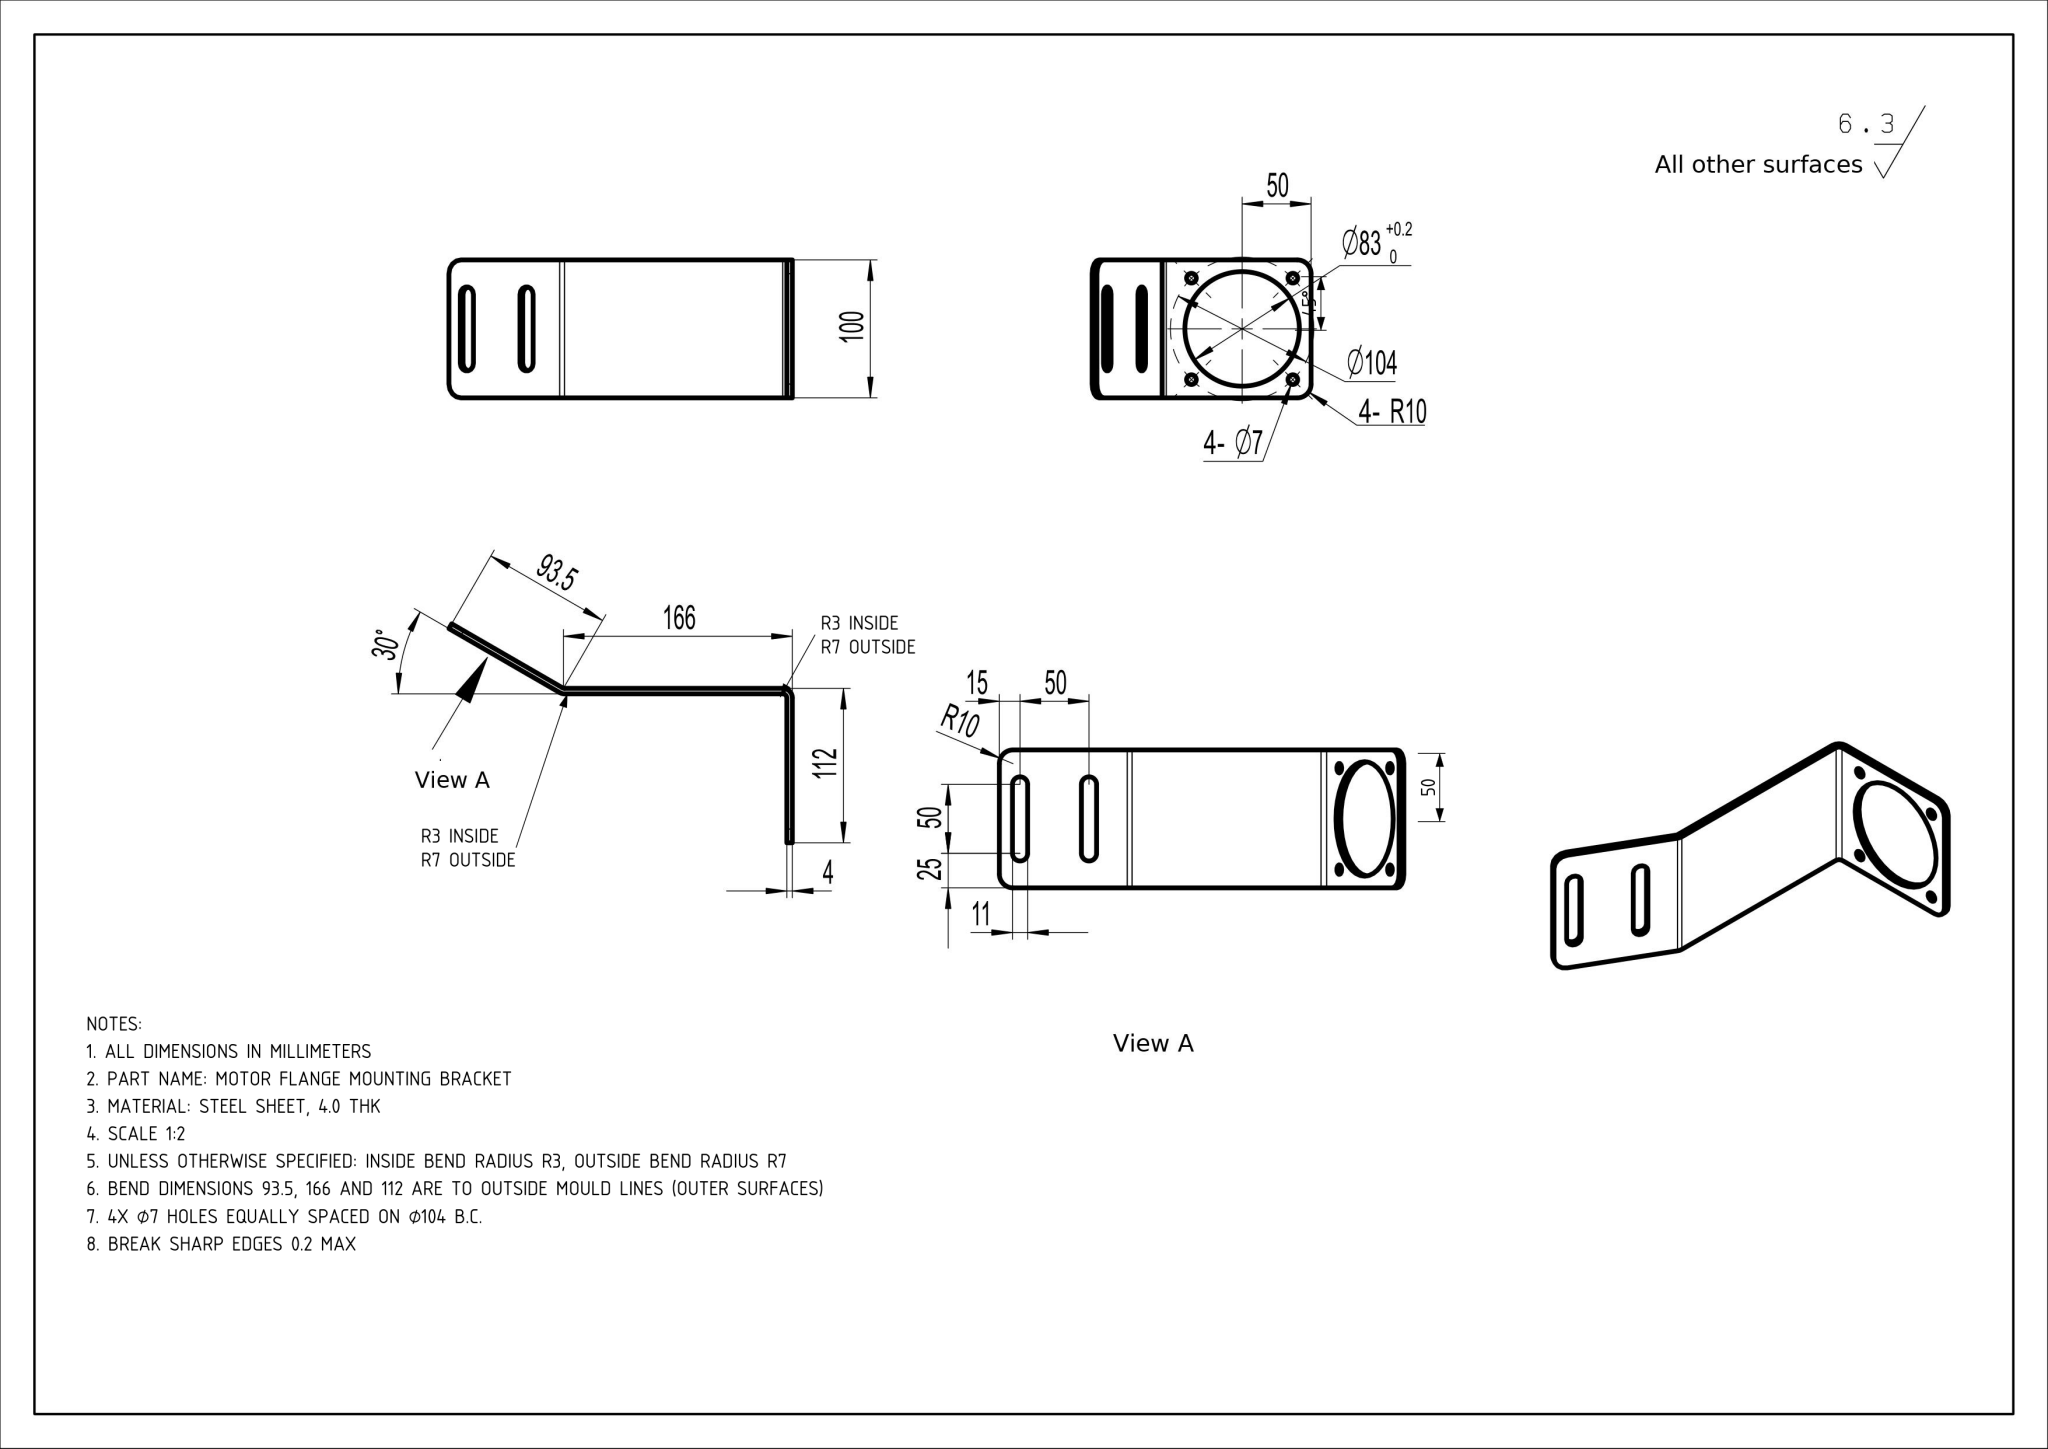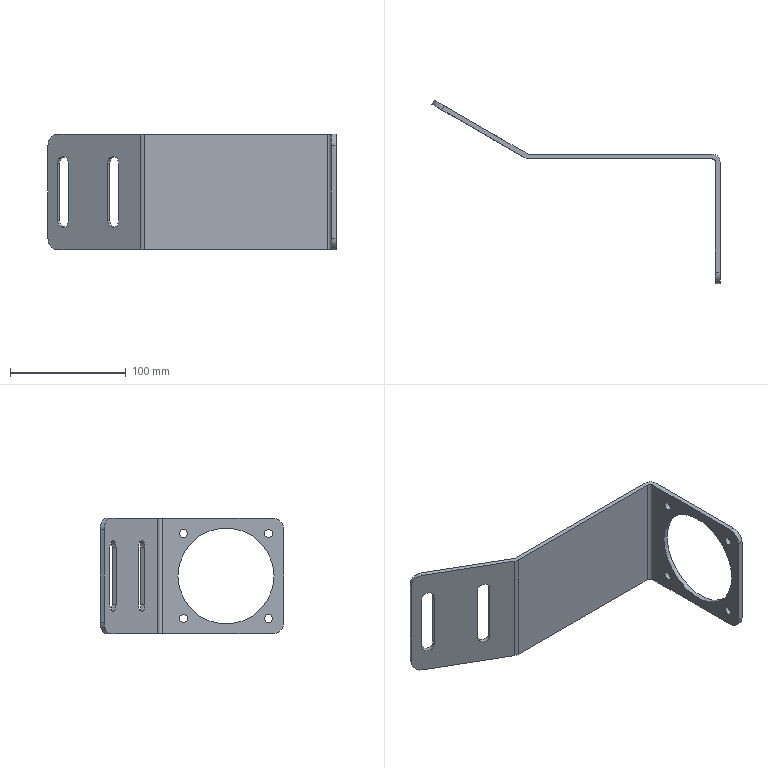Part | NX | mm | 1 solid | 31 faces | box 249.03 x 158.77 x 100 mm | volume 118808 mm3 | cylinder 17 | plane 14 | commonest cylinder face diameters 7 x4 11 x4 20 x4 14 x2 6 x2 83 x1
STEP:
#1=CARTESIAN_POINT('',(0.,0.,0.));
#2=DIRECTION('',(0.,0.,1.));
#3=DIRECTION('',(1.,0.,0.));
#4=AXIS2_PLACEMENT_3D('',#1,#2,#3);
#5=(LENGTH_UNIT()NAMED_UNIT(*)SI_UNIT(.MILLI.,.METRE.));
#6=UNCERTAINTY_MEASURE_WITH_UNIT(LENGTH_MEASURE(0.00002),#5,'','');
#7=(NAMED_UNIT(*)PLANE_ANGLE_UNIT()SI_UNIT($,.RADIAN.));
#8=PLANE_ANGLE_MEASURE_WITH_UNIT(PLANE_ANGLE_MEASURE(0.01745),#7);
#9=DIMENSIONAL_EXPONENTS(0.,0.,0.,0.,0.,0.,0.);
#10=(CONVERSION_BASED_UNIT('',#8)NAMED_UNIT(#9)PLANE_ANGLE_UNIT());
#11=(NAMED_UNIT(*)SI_UNIT($,.STERADIAN.)SOLID_ANGLE_UNIT());
#12=(GEOMETRIC_REPRESENTATION_CONTEXT(3)GLOBAL_UNCERTAINTY_ASSIGNED_CONTEXT((#6))GLOBAL_UNIT_ASSIGNED_CONTEXT((#5,#10,#11))REPRESENTATION_CONTEXT('',''));
#13=SHAPE_REPRESENTATION('',(#4),#12);
#14=CARTESIAN_POINT('',(4.,10.,0.));
#15=VERTEX_POINT('',#14);
#16=CARTESIAN_POINT('',(4.,105.,0.));
#17=VERTEX_POINT('',#16);
#18=CARTESIAN_POINT('',(4.,0.,0.));
#19=DIRECTION('',(0.,1.,0.));
#20=VECTOR('',#19,1.);
#21=LINE('',#18,#20);
#22=EDGE_CURVE('',#15,#17,#21,.T.);
#23=ORIENTED_EDGE('',*,*,#22,.F.);
#24=CARTESIAN_POINT('',(0.,10.,0.));
#25=VERTEX_POINT('',#24);
#26=CARTESIAN_POINT('',(4.,10.,0.));
#27=DIRECTION('',(-1.,0.,0.));
#28=VECTOR('',#27,1.);
#29=LINE('',#26,#28);
#30=EDGE_CURVE('',#15,#25,#29,.T.);
#31=ORIENTED_EDGE('',*,*,#30,.T.);
#32=CARTESIAN_POINT('',(0.,105.,0.));
#33=VERTEX_POINT('',#32);
#34=CARTESIAN_POINT('',(0.,0.,0.));
#35=DIRECTION('',(0.,1.,0.));
#36=VECTOR('',#35,1.);
#37=LINE('',#34,#36);
#38=EDGE_CURVE('',#25,#33,#37,.T.);
#39=ORIENTED_EDGE('',*,*,#38,.T.);
#40=CARTESIAN_POINT('',(-3.,108.,0.));
#41=VERTEX_POINT('',#40);
#42=CARTESIAN_POINT('',(-3.,105.,0.));
#43=DIRECTION('',(0.,0.,1.));
#44=DIRECTION('',(1.,0.,0.));
#45=AXIS2_PLACEMENT_3D('',#42,#43,#44);
#46=CIRCLE('',#45,3.);
#47=EDGE_CURVE('',#33,#41,#46,.T.);
#48=ORIENTED_EDGE('',*,*,#47,.T.);
#49=CARTESIAN_POINT('',(-161.214,108.,0.));
#50=VERTEX_POINT('',#49);
#51=CARTESIAN_POINT('',(108.786,108.,0.));
#52=DIRECTION('',(-1.,0.,0.));
#53=VECTOR('',#52,1.);
#54=LINE('',#51,#53);
#55=EDGE_CURVE('',#41,#50,#54,.T.);
#56=ORIENTED_EDGE('',*,*,#55,.T.);
#57=CARTESIAN_POINT('',(-164.714,108.938,0.));
#58=VERTEX_POINT('',#57);
#59=CARTESIAN_POINT('',(-161.214,115.,0.));
#60=DIRECTION('',(0.,-0.,-1.));
#61=DIRECTION('',(0.,1.,0.));
#62=AXIS2_PLACEMENT_3D('',#59,#60,#61);
#63=CIRCLE('',#62,7.);
#64=EDGE_CURVE('',#50,#58,#63,.T.);
#65=ORIENTED_EDGE('',*,*,#64,.T.);
#66=CARTESIAN_POINT('',(-236.367,150.307,0.));
#67=VERTEX_POINT('',#66);
#68=CARTESIAN_POINT('',(71.072,-27.193,0.));
#69=DIRECTION('',(-0.866,0.5,0.));
#70=VECTOR('',#69,1.);
#71=LINE('',#68,#70);
#72=EDGE_CURVE('',#58,#67,#71,.T.);
#73=ORIENTED_EDGE('',*,*,#72,.T.);
#74=CARTESIAN_POINT('',(-234.367,153.771,0.));
#75=VERTEX_POINT('',#74);
#76=CARTESIAN_POINT('',(-241.36,141.659,0.));
#77=DIRECTION('',(0.5,0.866,0.));
#78=VECTOR('',#77,1.);
#79=LINE('',#76,#78);
#80=EDGE_CURVE('',#67,#75,#79,.T.);
#81=ORIENTED_EDGE('',*,*,#80,.T.);
#82=CARTESIAN_POINT('',(-162.714,112.402,0.));
#83=VERTEX_POINT('',#82);
#84=CARTESIAN_POINT('',(73.072,-23.729,0.));
#85=DIRECTION('',(-0.866,0.5,0.));
#86=VECTOR('',#85,1.);
#87=LINE('',#84,#86);
#88=EDGE_CURVE('',#83,#75,#87,.T.);
#89=ORIENTED_EDGE('',*,*,#88,.F.);
#90=CARTESIAN_POINT('',(-161.214,112.,0.));
#91=VERTEX_POINT('',#90);
#92=CARTESIAN_POINT('',(-161.214,115.,0.));
#93=DIRECTION('',(0.,-0.,-1.));
#94=DIRECTION('',(-1.,0.,-0.));
#95=AXIS2_PLACEMENT_3D('',#92,#93,#94);
#96=CIRCLE('',#95,3.);
#97=EDGE_CURVE('',#91,#83,#96,.T.);
#98=ORIENTED_EDGE('',*,*,#97,.F.);
#99=CARTESIAN_POINT('',(-3.,112.,0.));
#100=VERTEX_POINT('',#99);
#101=CARTESIAN_POINT('',(108.786,112.,0.));
#102=DIRECTION('',(-1.,0.,0.));
#103=VECTOR('',#102,1.);
#104=LINE('',#101,#103);
#105=EDGE_CURVE('',#100,#91,#104,.T.);
#106=ORIENTED_EDGE('',*,*,#105,.F.);
#107=CARTESIAN_POINT('',(-3.,105.,0.));
#108=DIRECTION('',(0.,0.,1.));
#109=DIRECTION('',(-1.,0.,0.));
#110=AXIS2_PLACEMENT_3D('',#107,#108,#109);
#111=CIRCLE('',#110,7.);
#112=EDGE_CURVE('',#17,#100,#111,.T.);
#113=ORIENTED_EDGE('',*,*,#112,.F.);
#114=EDGE_LOOP('',(#23,#31,#39,#48,#56,#65,#73,#81,#89,#98,#106,#113));
#115=FACE_OUTER_BOUND('',#114,.T.);
#116=CARTESIAN_POINT('',(4.,0.,0.));
#117=DIRECTION('',(0.,0.,1.));
#118=DIRECTION('',(1.,0.,0.));
#119=AXIS2_PLACEMENT_3D('',#116,#117,#118);
#120=PLANE('',#119);
#121=ADVANCED_FACE('',(#115),#120,.F.);
#122=ORIENTED_EDGE('',*,*,#105,.T.);
#123=CARTESIAN_POINT('',(-161.214,112.,100.));
#124=VERTEX_POINT('',#123);
#125=CARTESIAN_POINT('',(-161.214,112.,-19.));
#126=DIRECTION('',(0.,0.,1.));
#127=VECTOR('',#126,1.);
#128=LINE('',#125,#127);
#129=EDGE_CURVE('',#91,#124,#128,.T.);
#130=ORIENTED_EDGE('',*,*,#129,.T.);
#131=CARTESIAN_POINT('',(-3.,112.,100.));
#132=VERTEX_POINT('',#131);
#133=CARTESIAN_POINT('',(-291.214,112.,100.));
#134=DIRECTION('',(1.,-0.,-0.));
#135=VECTOR('',#134,1.);
#136=LINE('',#133,#135);
#137=EDGE_CURVE('',#124,#132,#136,.T.);
#138=ORIENTED_EDGE('',*,*,#137,.T.);
#139=CARTESIAN_POINT('',(-3.,112.,-30.));
#140=DIRECTION('',(0.,-0.,1.));
#141=VECTOR('',#140,1.);
#142=LINE('',#139,#141);
#143=EDGE_CURVE('',#100,#132,#142,.T.);
#144=ORIENTED_EDGE('',*,*,#143,.F.);
#145=EDGE_LOOP('',(#122,#130,#138,#144));
#146=FACE_OUTER_BOUND('',#145,.T.);
#147=CARTESIAN_POINT('',(58.786,112.,50.));
#148=DIRECTION('',(0.,1.,0.));
#149=DIRECTION('',(0.,0.,-1.));
#150=AXIS2_PLACEMENT_3D('',#147,#148,#149);
#151=PLANE('',#150);
#152=ADVANCED_FACE('',(#146),#151,.T.);
#153=CARTESIAN_POINT('',(4.,83.27,13.23));
#154=VERTEX_POINT('',#153);
#155=CARTESIAN_POINT('',(4.,86.77,13.23));
#156=DIRECTION('',(1.,0.,0.));
#157=DIRECTION('',(0.,-1.,0.));
#158=AXIS2_PLACEMENT_3D('',#155,#156,#157);
#159=CIRCLE('',#158,3.5);
#160=EDGE_CURVE('',#154,#154,#159,.T.);
#161=ORIENTED_EDGE('',*,*,#160,.F.);
#162=EDGE_LOOP('',(#161));
#163=FACE_BOUND('',#162,.T.);
#164=CARTESIAN_POINT('',(4.,16.73,86.77));
#165=VERTEX_POINT('',#164);
#166=CARTESIAN_POINT('',(4.,13.23,86.77));
#167=DIRECTION('',(1.,0.,0.));
#168=DIRECTION('',(0.,1.,0.));
#169=AXIS2_PLACEMENT_3D('',#166,#167,#168);
#170=CIRCLE('',#169,3.5);
#171=EDGE_CURVE('',#165,#165,#170,.T.);
#172=ORIENTED_EDGE('',*,*,#171,.F.);
#173=EDGE_LOOP('',(#172));
#174=FACE_BOUND('',#173,.T.);
#175=CARTESIAN_POINT('',(4.,13.23,16.73));
#176=VERTEX_POINT('',#175);
#177=CARTESIAN_POINT('',(4.,13.23,13.23));
#178=DIRECTION('',(1.,0.,0.));
#179=DIRECTION('',(0.,0.,1.));
#180=AXIS2_PLACEMENT_3D('',#177,#178,#179);
#181=CIRCLE('',#180,3.5);
#182=EDGE_CURVE('',#176,#176,#181,.T.);
#183=ORIENTED_EDGE('',*,*,#182,.F.);
#184=EDGE_LOOP('',(#183));
#185=FACE_BOUND('',#184,.T.);
#186=CARTESIAN_POINT('',(4.,86.77,83.27));
#187=VERTEX_POINT('',#186);
#188=CARTESIAN_POINT('',(4.,86.77,86.77));
#189=DIRECTION('',(1.,0.,0.));
#190=DIRECTION('',(0.,0.,-1.));
#191=AXIS2_PLACEMENT_3D('',#188,#189,#190);
#192=CIRCLE('',#191,3.5);
#193=EDGE_CURVE('',#187,#187,#192,.T.);
#194=ORIENTED_EDGE('',*,*,#193,.F.);
#195=EDGE_LOOP('',(#194));
#196=FACE_BOUND('',#195,.T.);
#197=CARTESIAN_POINT('',(4.,91.5,50.));
#198=VERTEX_POINT('',#197);
#199=CARTESIAN_POINT('',(4.,50.,50.));
#200=DIRECTION('',(1.,0.,0.));
#201=DIRECTION('',(0.,1.,0.));
#202=AXIS2_PLACEMENT_3D('',#199,#200,#201);
#203=CIRCLE('',#202,41.5);
#204=EDGE_CURVE('',#198,#198,#203,.T.);
#205=ORIENTED_EDGE('',*,*,#204,.F.);
#206=EDGE_LOOP('',(#205));
#207=FACE_BOUND('',#206,.T.);
#208=CARTESIAN_POINT('',(4.,0.,90.));
#209=VERTEX_POINT('',#208);
#210=CARTESIAN_POINT('',(4.,0.,10.));
#211=VERTEX_POINT('',#210);
#212=CARTESIAN_POINT('',(4.,0.,100.));
#213=DIRECTION('',(0.,-0.,-1.));
#214=VECTOR('',#213,1.);
#215=LINE('',#212,#214);
#216=EDGE_CURVE('',#209,#211,#215,.T.);
#217=ORIENTED_EDGE('',*,*,#216,.T.);
#218=CARTESIAN_POINT('',(4.,10.,10.));
#219=DIRECTION('',(1.,0.,0.));
#220=DIRECTION('',(0.,0.,-1.));
#221=AXIS2_PLACEMENT_3D('',#218,#219,#220);
#222=CIRCLE('',#221,10.);
#223=EDGE_CURVE('',#211,#15,#222,.T.);
#224=ORIENTED_EDGE('',*,*,#223,.T.);
#225=ORIENTED_EDGE('',*,*,#22,.T.);
#226=CARTESIAN_POINT('',(4.,105.,100.));
#227=VERTEX_POINT('',#226);
#228=CARTESIAN_POINT('',(4.,105.,-30.));
#229=DIRECTION('',(0.,0.,-1.));
#230=VECTOR('',#229,1.);
#231=LINE('',#228,#230);
#232=EDGE_CURVE('',#227,#17,#231,.T.);
#233=ORIENTED_EDGE('',*,*,#232,.F.);
#234=CARTESIAN_POINT('',(4.,10.,100.));
#235=VERTEX_POINT('',#234);
#236=CARTESIAN_POINT('',(4.,400.,100.));
#237=DIRECTION('',(0.,-1.,-0.));
#238=VECTOR('',#237,1.);
#239=LINE('',#236,#238);
#240=EDGE_CURVE('',#227,#235,#239,.T.);
#241=ORIENTED_EDGE('',*,*,#240,.T.);
#242=CARTESIAN_POINT('',(4.,10.,90.));
#243=DIRECTION('',(1.,0.,0.));
#244=DIRECTION('',(0.,0.,-1.));
#245=AXIS2_PLACEMENT_3D('',#242,#243,#244);
#246=CIRCLE('',#245,10.);
#247=EDGE_CURVE('',#235,#209,#246,.T.);
#248=ORIENTED_EDGE('',*,*,#247,.T.);
#249=EDGE_LOOP('',(#217,#224,#225,#233,#241,#248));
#250=FACE_BOUND('',#249,.T.);
#251=CARTESIAN_POINT('',(4.,50.,50.));
#252=DIRECTION('',(1.,0.,0.));
#253=DIRECTION('',(0.,0.,-1.));
#254=AXIS2_PLACEMENT_3D('',#251,#252,#253);
#255=PLANE('',#254);
#256=ADVANCED_FACE('',(#163,#174,#185,#196,#207,#250),#255,.T.);
#257=CARTESIAN_POINT('',(0.,0.,90.));
#258=VERTEX_POINT('',#257);
#259=CARTESIAN_POINT('',(0.,0.,10.));
#260=VERTEX_POINT('',#259);
#261=CARTESIAN_POINT('',(0.,0.,100.));
#262=DIRECTION('',(0.,-0.,-1.));
#263=VECTOR('',#262,1.);
#264=LINE('',#261,#263);
#265=EDGE_CURVE('',#258,#260,#264,.T.);
#266=ORIENTED_EDGE('',*,*,#265,.T.);
#267=CARTESIAN_POINT('',(4.,0.,10.));
#268=DIRECTION('',(1.,0.,0.));
#269=VECTOR('',#268,1.);
#270=LINE('',#267,#269);
#271=EDGE_CURVE('',#260,#211,#270,.T.);
#272=ORIENTED_EDGE('',*,*,#271,.T.);
#273=ORIENTED_EDGE('',*,*,#216,.F.);
#274=CARTESIAN_POINT('',(4.,0.,90.));
#275=DIRECTION('',(-1.,0.,0.));
#276=VECTOR('',#275,1.);
#277=LINE('',#274,#276);
#278=EDGE_CURVE('',#209,#258,#277,.T.);
#279=ORIENTED_EDGE('',*,*,#278,.T.);
#280=EDGE_LOOP('',(#266,#272,#273,#279));
#281=FACE_OUTER_BOUND('',#280,.T.);
#282=CARTESIAN_POINT('',(4.,0.,100.));
#283=DIRECTION('',(0.,1.,-0.));
#284=DIRECTION('',(0.,0.,1.));
#285=AXIS2_PLACEMENT_3D('',#282,#283,#284);
#286=PLANE('',#285);
#287=ADVANCED_FACE('',(#281),#286,.F.);
#288=CARTESIAN_POINT('',(0.,105.,100.));
#289=VERTEX_POINT('',#288);
#290=CARTESIAN_POINT('',(0.,10.,100.));
#291=VERTEX_POINT('',#290);
#292=CARTESIAN_POINT('',(0.,400.,100.));
#293=DIRECTION('',(0.,-1.,-0.));
#294=VECTOR('',#293,1.);
#295=LINE('',#292,#294);
#296=EDGE_CURVE('',#289,#291,#295,.T.);
#297=ORIENTED_EDGE('',*,*,#296,.T.);
#298=CARTESIAN_POINT('',(4.,10.,100.));
#299=DIRECTION('',(1.,0.,0.));
#300=VECTOR('',#299,1.);
#301=LINE('',#298,#300);
#302=EDGE_CURVE('',#291,#235,#301,.T.);
#303=ORIENTED_EDGE('',*,*,#302,.T.);
#304=ORIENTED_EDGE('',*,*,#240,.F.);
#305=CARTESIAN_POINT('',(-3.,105.,100.));
#306=DIRECTION('',(0.,0.,-1.));
#307=DIRECTION('',(-1.,0.,0.));
#308=AXIS2_PLACEMENT_3D('',#305,#306,#307);
#309=CIRCLE('',#308,7.);
#310=EDGE_CURVE('',#132,#227,#309,.T.);
#311=ORIENTED_EDGE('',*,*,#310,.F.);
#312=ORIENTED_EDGE('',*,*,#137,.F.);
#313=CARTESIAN_POINT('',(-162.714,112.402,100.));
#314=VERTEX_POINT('',#313);
#315=CARTESIAN_POINT('',(-161.214,115.,100.));
#316=DIRECTION('',(-0.,0.,1.));
#317=DIRECTION('',(-1.,0.,0.));
#318=AXIS2_PLACEMENT_3D('',#315,#316,#317);
#319=CIRCLE('',#318,3.);
#320=EDGE_CURVE('',#314,#124,#319,.T.);
#321=ORIENTED_EDGE('',*,*,#320,.F.);
#322=CARTESIAN_POINT('',(-234.367,153.771,100.));
#323=VERTEX_POINT('',#322);
#324=CARTESIAN_POINT('',(-273.339,176.271,100.));
#325=DIRECTION('',(0.866,-0.5,-0.));
#326=VECTOR('',#325,1.);
#327=LINE('',#324,#326);
#328=EDGE_CURVE('',#323,#314,#327,.T.);
#329=ORIENTED_EDGE('',*,*,#328,.F.);
#330=CARTESIAN_POINT('',(-236.367,150.307,100.));
#331=VERTEX_POINT('',#330);
#332=CARTESIAN_POINT('',(-68.155,441.659,100.));
#333=DIRECTION('',(-0.5,-0.866,-0.));
#334=VECTOR('',#333,1.);
#335=LINE('',#332,#334);
#336=EDGE_CURVE('',#323,#331,#335,.T.);
#337=ORIENTED_EDGE('',*,*,#336,.T.);
#338=CARTESIAN_POINT('',(-164.714,108.938,100.));
#339=VERTEX_POINT('',#338);
#340=CARTESIAN_POINT('',(-275.339,172.807,100.));
#341=DIRECTION('',(0.866,-0.5,-0.));
#342=VECTOR('',#341,1.);
#343=LINE('',#340,#342);
#344=EDGE_CURVE('',#331,#339,#343,.T.);
#345=ORIENTED_EDGE('',*,*,#344,.T.);
#346=CARTESIAN_POINT('',(-161.214,108.,100.));
#347=VERTEX_POINT('',#346);
#348=CARTESIAN_POINT('',(-161.214,115.,100.));
#349=DIRECTION('',(-0.,0.,1.));
#350=DIRECTION('',(0.,1.,0.));
#351=AXIS2_PLACEMENT_3D('',#348,#349,#350);
#352=CIRCLE('',#351,7.);
#353=EDGE_CURVE('',#339,#347,#352,.T.);
#354=ORIENTED_EDGE('',*,*,#353,.T.);
#355=CARTESIAN_POINT('',(-3.,108.,100.));
#356=VERTEX_POINT('',#355);
#357=CARTESIAN_POINT('',(-291.214,108.,100.));
#358=DIRECTION('',(1.,-0.,-0.));
#359=VECTOR('',#358,1.);
#360=LINE('',#357,#359);
#361=EDGE_CURVE('',#347,#356,#360,.T.);
#362=ORIENTED_EDGE('',*,*,#361,.T.);
#363=CARTESIAN_POINT('',(-3.,105.,100.));
#364=DIRECTION('',(0.,0.,-1.));
#365=DIRECTION('',(1.,0.,0.));
#366=AXIS2_PLACEMENT_3D('',#363,#364,#365);
#367=CIRCLE('',#366,3.);
#368=EDGE_CURVE('',#356,#289,#367,.T.);
#369=ORIENTED_EDGE('',*,*,#368,.T.);
#370=EDGE_LOOP('',(#297,#303,#304,#311,#312,#321,#329,#337,#345,#354,#362,#369));
#371=FACE_OUTER_BOUND('',#370,.T.);
#372=CARTESIAN_POINT('',(4.,400.,100.));
#373=DIRECTION('',(0.,0.,-1.));
#374=DIRECTION('',(0.,1.,0.));
#375=AXIS2_PLACEMENT_3D('',#372,#373,#374);
#376=PLANE('',#375);
#377=ADVANCED_FACE('',(#371),#376,.F.);
#378=ORIENTED_EDGE('',*,*,#204,.T.);
#379=EDGE_LOOP('',(#378));
#380=FACE_BOUND('',#379,.T.);
#381=CARTESIAN_POINT('',(0.,91.5,50.));
#382=VERTEX_POINT('',#381);
#383=CARTESIAN_POINT('',(0.,50.,50.));
#384=DIRECTION('',(1.,0.,0.));
#385=DIRECTION('',(0.,1.,0.));
#386=AXIS2_PLACEMENT_3D('',#383,#384,#385);
#387=CIRCLE('',#386,41.5);
#388=EDGE_CURVE('',#382,#382,#387,.T.);
#389=ORIENTED_EDGE('',*,*,#388,.F.);
#390=EDGE_LOOP('',(#389));
#391=FACE_BOUND('',#390,.T.);
#392=CARTESIAN_POINT('',(4.,50.,50.));
#393=DIRECTION('',(-1.,0.,0.));
#394=DIRECTION('',(0.,0.,1.));
#395=AXIS2_PLACEMENT_3D('',#392,#393,#394);
#396=CYLINDRICAL_SURFACE('',#395,41.5);
#397=ADVANCED_FACE('',(#380,#391),#396,.F.);
#398=ORIENTED_EDGE('',*,*,#38,.F.);
#399=CARTESIAN_POINT('',(0.,10.,10.));
#400=DIRECTION('',(-1.,0.,0.));
#401=DIRECTION('',(0.,0.,-1.));
#402=AXIS2_PLACEMENT_3D('',#399,#400,#401);
#403=CIRCLE('',#402,10.);
#404=EDGE_CURVE('',#25,#260,#403,.T.);
#405=ORIENTED_EDGE('',*,*,#404,.T.);
#406=ORIENTED_EDGE('',*,*,#265,.F.);
#407=CARTESIAN_POINT('',(0.,10.,90.));
#408=DIRECTION('',(-1.,0.,0.));
#409=DIRECTION('',(0.,0.,-1.));
#410=AXIS2_PLACEMENT_3D('',#407,#408,#409);
#411=CIRCLE('',#410,10.);
#412=EDGE_CURVE('',#258,#291,#411,.T.);
#413=ORIENTED_EDGE('',*,*,#412,.T.);
#414=ORIENTED_EDGE('',*,*,#296,.F.);
#415=CARTESIAN_POINT('',(0.,105.,-30.));
#416=DIRECTION('',(0.,-0.,1.));
#417=VECTOR('',#416,1.);
#418=LINE('',#415,#417);
#419=EDGE_CURVE('',#33,#289,#418,.T.);
#420=ORIENTED_EDGE('',*,*,#419,.F.);
#421=EDGE_LOOP('',(#398,#405,#406,#413,#414,#420));
#422=FACE_BOUND('',#421,.T.);
#423=CARTESIAN_POINT('',(0.,83.27,13.23));
#424=VERTEX_POINT('',#423);
#425=CARTESIAN_POINT('',(0.,86.77,13.23));
#426=DIRECTION('',(1.,0.,0.));
#427=DIRECTION('',(0.,-1.,0.));
#428=AXIS2_PLACEMENT_3D('',#425,#426,#427);
#429=CIRCLE('',#428,3.5);
#430=EDGE_CURVE('',#424,#424,#429,.T.);
#431=ORIENTED_EDGE('',*,*,#430,.T.);
#432=EDGE_LOOP('',(#431));
#433=FACE_BOUND('',#432,.T.);
#434=CARTESIAN_POINT('',(0.,16.73,86.77));
#435=VERTEX_POINT('',#434);
#436=CARTESIAN_POINT('',(0.,13.23,86.77));
#437=DIRECTION('',(1.,0.,0.));
#438=DIRECTION('',(0.,1.,0.));
#439=AXIS2_PLACEMENT_3D('',#436,#437,#438);
#440=CIRCLE('',#439,3.5);
#441=EDGE_CURVE('',#435,#435,#440,.T.);
#442=ORIENTED_EDGE('',*,*,#441,.T.);
#443=EDGE_LOOP('',(#442));
#444=FACE_BOUND('',#443,.T.);
#445=CARTESIAN_POINT('',(0.,13.23,16.73));
#446=VERTEX_POINT('',#445);
#447=CARTESIAN_POINT('',(0.,13.23,13.23));
#448=DIRECTION('',(1.,0.,0.));
#449=DIRECTION('',(0.,0.,1.));
#450=AXIS2_PLACEMENT_3D('',#447,#448,#449);
#451=CIRCLE('',#450,3.5);
#452=EDGE_CURVE('',#446,#446,#451,.T.);
#453=ORIENTED_EDGE('',*,*,#452,.T.);
#454=EDGE_LOOP('',(#453));
#455=FACE_BOUND('',#454,.T.);
#456=CARTESIAN_POINT('',(0.,86.77,83.27));
#457=VERTEX_POINT('',#456);
#458=CARTESIAN_POINT('',(0.,86.77,86.77));
#459=DIRECTION('',(1.,0.,0.));
#460=DIRECTION('',(0.,0.,-1.));
#461=AXIS2_PLACEMENT_3D('',#458,#459,#460);
#462=CIRCLE('',#461,3.5);
#463=EDGE_CURVE('',#457,#457,#462,.T.);
#464=ORIENTED_EDGE('',*,*,#463,.T.);
#465=EDGE_LOOP('',(#464));
#466=FACE_BOUND('',#465,.T.);
#467=ORIENTED_EDGE('',*,*,#388,.T.);
#468=EDGE_LOOP('',(#467));
#469=FACE_BOUND('',#468,.T.);
#470=CARTESIAN_POINT('',(0.,50.,50.));
#471=DIRECTION('',(1.,0.,0.));
#472=DIRECTION('',(0.,0.,-1.));
#473=AXIS2_PLACEMENT_3D('',#470,#471,#472);
#474=PLANE('',#473);
#475=ADVANCED_FACE('',(#422,#433,#444,#455,#466,#469),#474,.F.);
#476=ORIENTED_EDGE('',*,*,#463,.F.);
#477=EDGE_LOOP('',(#476));
#478=FACE_BOUND('',#477,.T.);
#479=ORIENTED_EDGE('',*,*,#193,.T.);
#480=EDGE_LOOP('',(#479));
#481=FACE_BOUND('',#480,.T.);
#482=CARTESIAN_POINT('',(0.,86.77,86.77));
#483=DIRECTION('',(1.,0.,0.));
#484=DIRECTION('',(0.,0.,-1.));
#485=AXIS2_PLACEMENT_3D('',#482,#483,#484);
#486=CYLINDRICAL_SURFACE('',#485,3.5);
#487=ADVANCED_FACE('',(#478,#481),#486,.F.);
#488=ORIENTED_EDGE('',*,*,#452,.F.);
#489=EDGE_LOOP('',(#488));
#490=FACE_BOUND('',#489,.T.);
#491=ORIENTED_EDGE('',*,*,#182,.T.);
#492=EDGE_LOOP('',(#491));
#493=FACE_BOUND('',#492,.T.);
#494=CARTESIAN_POINT('',(0.,13.23,13.23));
#495=DIRECTION('',(1.,0.,0.));
#496=DIRECTION('',(0.,0.,-1.));
#497=AXIS2_PLACEMENT_3D('',#494,#495,#496);
#498=CYLINDRICAL_SURFACE('',#497,3.5);
#499=ADVANCED_FACE('',(#490,#493),#498,.F.);
#500=ORIENTED_EDGE('',*,*,#441,.F.);
#501=EDGE_LOOP('',(#500));
#502=FACE_BOUND('',#501,.T.);
#503=ORIENTED_EDGE('',*,*,#171,.T.);
#504=EDGE_LOOP('',(#503));
#505=FACE_BOUND('',#504,.T.);
#506=CARTESIAN_POINT('',(0.,13.23,86.77));
#507=DIRECTION('',(1.,0.,0.));
#508=DIRECTION('',(0.,0.,-1.));
#509=AXIS2_PLACEMENT_3D('',#506,#507,#508);
#510=CYLINDRICAL_SURFACE('',#509,3.5);
#511=ADVANCED_FACE('',(#502,#505),#510,.F.);
#512=ORIENTED_EDGE('',*,*,#430,.F.);
#513=EDGE_LOOP('',(#512));
#514=FACE_BOUND('',#513,.T.);
#515=ORIENTED_EDGE('',*,*,#160,.T.);
#516=EDGE_LOOP('',(#515));
#517=FACE_BOUND('',#516,.T.);
#518=CARTESIAN_POINT('',(0.,86.77,13.23));
#519=DIRECTION('',(1.,0.,0.));
#520=DIRECTION('',(0.,0.,-1.));
#521=AXIS2_PLACEMENT_3D('',#518,#519,#520);
#522=CYLINDRICAL_SURFACE('',#521,3.5);
#523=ADVANCED_FACE('',(#514,#517),#522,.F.);
#524=CARTESIAN_POINT('',(-161.214,108.,-19.));
#525=DIRECTION('',(0.,0.,1.));
#526=VECTOR('',#525,1.);
#527=LINE('',#524,#526);
#528=EDGE_CURVE('',#50,#347,#527,.T.);
#529=ORIENTED_EDGE('',*,*,#528,.F.);
#530=ORIENTED_EDGE('',*,*,#55,.F.);
#531=CARTESIAN_POINT('',(-3.,108.,-30.));
#532=DIRECTION('',(-0.,0.,-1.));
#533=VECTOR('',#532,1.);
#534=LINE('',#531,#533);
#535=EDGE_CURVE('',#356,#41,#534,.T.);
#536=ORIENTED_EDGE('',*,*,#535,.F.);
#537=ORIENTED_EDGE('',*,*,#361,.F.);
#538=EDGE_LOOP('',(#529,#530,#536,#537));
#539=FACE_OUTER_BOUND('',#538,.T.);
#540=CARTESIAN_POINT('',(58.786,108.,50.));
#541=DIRECTION('',(0.,1.,0.));
#542=DIRECTION('',(0.,0.,-1.));
#543=AXIS2_PLACEMENT_3D('',#540,#541,#542);
#544=PLANE('',#543);
#545=ADVANCED_FACE('',(#539),#544,.F.);
#546=ORIENTED_EDGE('',*,*,#232,.T.);
#547=ORIENTED_EDGE('',*,*,#112,.T.);
#548=ORIENTED_EDGE('',*,*,#143,.T.);
#549=ORIENTED_EDGE('',*,*,#310,.T.);
#550=EDGE_LOOP('',(#546,#547,#548,#549));
#551=FACE_OUTER_BOUND('',#550,.T.);
#552=CARTESIAN_POINT('',(-3.,105.,0.));
#553=DIRECTION('',(0.,0.,1.));
#554=DIRECTION('',(-1.,0.,0.));
#555=AXIS2_PLACEMENT_3D('',#552,#553,#554);
#556=CYLINDRICAL_SURFACE('',#555,7.);
#557=ADVANCED_FACE('',(#551),#556,.T.);
#558=ORIENTED_EDGE('',*,*,#419,.T.);
#559=ORIENTED_EDGE('',*,*,#368,.F.);
#560=ORIENTED_EDGE('',*,*,#535,.T.);
#561=ORIENTED_EDGE('',*,*,#47,.F.);
#562=EDGE_LOOP('',(#558,#559,#560,#561));
#563=FACE_OUTER_BOUND('',#562,.T.);
#564=CARTESIAN_POINT('',(-3.,105.,0.));
#565=DIRECTION('',(0.,0.,1.));
#566=DIRECTION('',(-1.,0.,0.));
#567=AXIS2_PLACEMENT_3D('',#564,#565,#566);
#568=CYLINDRICAL_SURFACE('',#567,3.);
#569=ADVANCED_FACE('',(#563),#568,.F.);
#570=CARTESIAN_POINT('',(-243.028,158.771,10.));
#571=VERTEX_POINT('',#570);
#572=CARTESIAN_POINT('',(-243.028,158.771,90.));
#573=VERTEX_POINT('',#572);
#574=CARTESIAN_POINT('',(-243.028,158.771,0.));
#575=DIRECTION('',(0.,0.,1.));
#576=VECTOR('',#575,1.);
#577=LINE('',#574,#576);
#578=EDGE_CURVE('',#571,#573,#577,.T.);
#579=ORIENTED_EDGE('',*,*,#578,.F.);
#580=CARTESIAN_POINT('',(-245.028,155.307,10.));
#581=VERTEX_POINT('',#580);
#582=CARTESIAN_POINT('',(-243.028,158.771,10.));
#583=DIRECTION('',(-0.5,-0.866,0.));
#584=VECTOR('',#583,1.);
#585=LINE('',#582,#584);
#586=EDGE_CURVE('',#571,#581,#585,.T.);
#587=ORIENTED_EDGE('',*,*,#586,.T.);
#588=CARTESIAN_POINT('',(-245.028,155.307,90.));
#589=VERTEX_POINT('',#588);
#590=CARTESIAN_POINT('',(-245.028,155.307,0.));
#591=DIRECTION('',(0.,0.,1.));
#592=VECTOR('',#591,1.);
#593=LINE('',#590,#592);
#594=EDGE_CURVE('',#581,#589,#593,.T.);
#595=ORIENTED_EDGE('',*,*,#594,.T.);
#596=CARTESIAN_POINT('',(-243.028,158.771,90.));
#597=DIRECTION('',(0.5,0.866,0.));
#598=VECTOR('',#597,1.);
#599=LINE('',#596,#598);
#600=EDGE_CURVE('',#589,#573,#599,.T.);
#601=ORIENTED_EDGE('',*,*,#600,.T.);
#602=EDGE_LOOP('',(#579,#587,#595,#601));
#603=FACE_OUTER_BOUND('',#602,.T.);
#604=CARTESIAN_POINT('',(-243.028,158.771,0.));
#605=DIRECTION('',(0.866,-0.5,0.));
#606=DIRECTION('',(0.,0.,-1.));
#607=AXIS2_PLACEMENT_3D('',#604,#605,#606);
#608=PLANE('',#607);
#609=ADVANCED_FACE('',(#603),#608,.F.);
#610=CARTESIAN_POINT('',(-193.499,125.557,75.));
#611=VERTEX_POINT('',#610);
#612=CARTESIAN_POINT('',(-193.499,125.557,25.));
#613=VERTEX_POINT('',#612);
#614=CARTESIAN_POINT('',(-193.499,125.557,50.));
#615=DIRECTION('',(0.,-0.,-1.));
#616=VECTOR('',#615,1.);
#617=LINE('',#614,#616);
#618=EDGE_CURVE('',#611,#613,#617,.T.);
#619=ORIENTED_EDGE('',*,*,#618,.F.);
#620=CARTESIAN_POINT('',(-183.973,120.057,75.));
#621=VERTEX_POINT('',#620);
#622=CARTESIAN_POINT('',(-188.736,122.807,75.));
#623=DIRECTION('',(-0.5,-0.866,0.));
#624=DIRECTION('',(-0.866,0.5,0.));
#625=AXIS2_PLACEMENT_3D('',#622,#623,#624);
#626=CIRCLE('',#625,5.5);
#627=EDGE_CURVE('',#621,#611,#626,.T.);
#628=ORIENTED_EDGE('',*,*,#627,.F.);
#629=CARTESIAN_POINT('',(-183.973,120.057,25.));
#630=VERTEX_POINT('',#629);
#631=CARTESIAN_POINT('',(-183.973,120.057,50.));
#632=DIRECTION('',(0.,0.,1.));
#633=VECTOR('',#632,1.);
#634=LINE('',#631,#633);
#635=EDGE_CURVE('',#630,#621,#634,.T.);
#636=ORIENTED_EDGE('',*,*,#635,.F.);
#637=CARTESIAN_POINT('',(-188.736,122.807,25.));
#638=DIRECTION('',(-0.5,-0.866,0.));
#639=DIRECTION('',(-0.866,0.5,0.));
#640=AXIS2_PLACEMENT_3D('',#637,#638,#639);
#641=CIRCLE('',#640,5.5);
#642=EDGE_CURVE('',#613,#630,#641,.T.);
#643=ORIENTED_EDGE('',*,*,#642,.F.);
#644=EDGE_LOOP('',(#619,#628,#636,#643));
#645=FACE_BOUND('',#644,.T.);
#646=CARTESIAN_POINT('',(-236.8,150.557,75.));
#647=VERTEX_POINT('',#646);
#648=CARTESIAN_POINT('',(-236.8,150.557,25.));
#649=VERTEX_POINT('',#648);
#650=CARTESIAN_POINT('',(-236.8,150.557,50.));
#651=DIRECTION('',(0.,-0.,-1.));
#652=VECTOR('',#651,1.);
#653=LINE('',#650,#652);
#654=EDGE_CURVE('',#647,#649,#653,.T.);
#655=ORIENTED_EDGE('',*,*,#654,.F.);
#656=CARTESIAN_POINT('',(-227.274,145.057,75.));
#657=VERTEX_POINT('',#656);
#658=CARTESIAN_POINT('',(-232.037,147.807,75.));
#659=DIRECTION('',(-0.5,-0.866,0.));
#660=DIRECTION('',(-0.866,0.5,0.));
#661=AXIS2_PLACEMENT_3D('',#658,#659,#660);
#662=CIRCLE('',#661,5.5);
#663=EDGE_CURVE('',#657,#647,#662,.T.);
#664=ORIENTED_EDGE('',*,*,#663,.F.);
#665=CARTESIAN_POINT('',(-227.274,145.057,25.));
#666=VERTEX_POINT('',#665);
#667=CARTESIAN_POINT('',(-227.274,145.057,50.));
#668=DIRECTION('',(-0.,0.,1.));
#669=VECTOR('',#668,1.);
#670=LINE('',#667,#669);
#671=EDGE_CURVE('',#666,#657,#670,.T.);
#672=ORIENTED_EDGE('',*,*,#671,.F.);
#673=CARTESIAN_POINT('',(-232.037,147.807,25.));
#674=DIRECTION('',(-0.5,-0.866,0.));
#675=DIRECTION('',(-0.866,0.5,0.));
#676=AXIS2_PLACEMENT_3D('',#673,#674,#675);
#677=CIRCLE('',#676,5.5);
#678=EDGE_CURVE('',#649,#666,#677,.T.);
#679=ORIENTED_EDGE('',*,*,#678,.F.);
#680=EDGE_LOOP('',(#655,#664,#672,#679));
#681=FACE_BOUND('',#680,.T.);
#682=ORIENTED_EDGE('',*,*,#594,.F.);
#683=CARTESIAN_POINT('',(-236.367,150.307,10.));
#684=DIRECTION('',(-0.5,-0.866,0.));
#685=DIRECTION('',(-0.866,0.5,0.));
#686=AXIS2_PLACEMENT_3D('',#683,#684,#685);
#687=CIRCLE('',#686,10.);
#688=EDGE_CURVE('',#581,#67,#687,.T.);
#689=ORIENTED_EDGE('',*,*,#688,.T.);
#690=ORIENTED_EDGE('',*,*,#72,.F.);
#691=CARTESIAN_POINT('',(-164.714,108.938,-19.));
#692=DIRECTION('',(-0.,-0.,-1.));
#693=VECTOR('',#692,1.);
#694=LINE('',#691,#693);
#695=EDGE_CURVE('',#339,#58,#694,.T.);
#696=ORIENTED_EDGE('',*,*,#695,.F.);
#697=ORIENTED_EDGE('',*,*,#344,.F.);
#698=CARTESIAN_POINT('',(-236.367,150.307,90.));
#699=DIRECTION('',(-0.5,-0.866,0.));
#700=DIRECTION('',(-0.866,0.5,0.));
#701=AXIS2_PLACEMENT_3D('',#698,#699,#700);
#702=CIRCLE('',#701,10.);
#703=EDGE_CURVE('',#331,#589,#702,.T.);
#704=ORIENTED_EDGE('',*,*,#703,.T.);
#705=EDGE_LOOP('',(#682,#689,#690,#696,#697,#704));
#706=FACE_BOUND('',#705,.T.);
#707=CARTESIAN_POINT('',(27.77,-2.193,50.));
#708=DIRECTION('',(0.5,0.866,0.));
#709=DIRECTION('',(0.,0.,-1.));
#710=AXIS2_PLACEMENT_3D('',#707,#708,#709);
#711=PLANE('',#710);
#712=ADVANCED_FACE('',(#645,#681,#706),#711,.F.);
#713=CARTESIAN_POINT('',(-181.973,123.521,75.));
#714=VERTEX_POINT('',#713);
#715=CARTESIAN_POINT('',(-191.499,129.021,75.));
#716=VERTEX_POINT('',#715);
#717=CARTESIAN_POINT('',(-186.736,126.271,75.));
#718=DIRECTION('',(-0.5,-0.866,0.));
#719=DIRECTION('',(-0.866,0.5,0.));
#720=AXIS2_PLACEMENT_3D('',#717,#718,#719);
#721=CIRCLE('',#720,5.5);
#722=EDGE_CURVE('',#714,#716,#721,.T.);
#723=ORIENTED_EDGE('',*,*,#722,.T.);
#724=CARTESIAN_POINT('',(-191.499,129.021,25.));
#725=VERTEX_POINT('',#724);
#726=CARTESIAN_POINT('',(-191.499,129.021,50.));
#727=DIRECTION('',(0.,-0.,-1.));
#728=VECTOR('',#727,1.);
#729=LINE('',#726,#728);
#730=EDGE_CURVE('',#716,#725,#729,.T.);
#731=ORIENTED_EDGE('',*,*,#730,.T.);
#732=CARTESIAN_POINT('',(-181.973,123.521,25.));
#733=VERTEX_POINT('',#732);
#734=CARTESIAN_POINT('',(-186.736,126.271,25.));
#735=DIRECTION('',(-0.5,-0.866,0.));
#736=DIRECTION('',(-0.866,0.5,0.));
#737=AXIS2_PLACEMENT_3D('',#734,#735,#736);
#738=CIRCLE('',#737,5.5);
#739=EDGE_CURVE('',#725,#733,#738,.T.);
#740=ORIENTED_EDGE('',*,*,#739,.T.);
#741=CARTESIAN_POINT('',(-181.973,123.521,50.));
#742=DIRECTION('',(0.,0.,1.));
#743=VECTOR('',#742,1.);
#744=LINE('',#741,#743);
#745=EDGE_CURVE('',#733,#714,#744,.T.);
#746=ORIENTED_EDGE('',*,*,#745,.T.);
#747=EDGE_LOOP('',(#723,#731,#740,#746));
#748=FACE_BOUND('',#747,.T.);
#749=CARTESIAN_POINT('',(-225.274,148.521,75.));
#750=VERTEX_POINT('',#749);
#751=CARTESIAN_POINT('',(-234.8,154.021,75.));
#752=VERTEX_POINT('',#751);
#753=CARTESIAN_POINT('',(-230.037,151.271,75.));
#754=DIRECTION('',(-0.5,-0.866,0.));
#755=DIRECTION('',(-0.866,0.5,0.));
#756=AXIS2_PLACEMENT_3D('',#753,#754,#755);
#757=CIRCLE('',#756,5.5);
#758=EDGE_CURVE('',#750,#752,#757,.T.);
#759=ORIENTED_EDGE('',*,*,#758,.T.);
#760=CARTESIAN_POINT('',(-234.8,154.021,25.));
#761=VERTEX_POINT('',#760);
#762=CARTESIAN_POINT('',(-234.8,154.021,50.));
#763=DIRECTION('',(0.,-0.,-1.));
#764=VECTOR('',#763,1.);
#765=LINE('',#762,#764);
#766=EDGE_CURVE('',#752,#761,#765,.T.);
#767=ORIENTED_EDGE('',*,*,#766,.T.);
#768=CARTESIAN_POINT('',(-225.274,148.521,25.));
#769=VERTEX_POINT('',#768);
#770=CARTESIAN_POINT('',(-230.037,151.271,25.));
#771=DIRECTION('',(-0.5,-0.866,0.));
#772=DIRECTION('',(-0.866,0.5,0.));
#773=AXIS2_PLACEMENT_3D('',#770,#771,#772);
#774=CIRCLE('',#773,5.5);
#775=EDGE_CURVE('',#761,#769,#774,.T.);
#776=ORIENTED_EDGE('',*,*,#775,.T.);
#777=CARTESIAN_POINT('',(-225.274,148.521,50.));
#778=DIRECTION('',(-0.,0.,1.));
#779=VECTOR('',#778,1.);
#780=LINE('',#777,#779);
#781=EDGE_CURVE('',#769,#750,#780,.T.);
#782=ORIENTED_EDGE('',*,*,#781,.T.);
#783=EDGE_LOOP('',(#759,#767,#776,#782));
#784=FACE_BOUND('',#783,.T.);
#785=ORIENTED_EDGE('',*,*,#88,.T.);
#786=CARTESIAN_POINT('',(-234.367,153.771,10.));
#787=DIRECTION('',(0.5,0.866,0.));
#788=DIRECTION('',(-0.866,0.5,0.));
#789=AXIS2_PLACEMENT_3D('',#786,#787,#788);
#790=CIRCLE('',#789,10.);
#791=EDGE_CURVE('',#75,#571,#790,.T.);
#792=ORIENTED_EDGE('',*,*,#791,.T.);
#793=ORIENTED_EDGE('',*,*,#578,.T.);
#794=CARTESIAN_POINT('',(-234.367,153.771,90.));
#795=DIRECTION('',(0.5,0.866,0.));
#796=DIRECTION('',(-0.866,0.5,0.));
#797=AXIS2_PLACEMENT_3D('',#794,#795,#796);
#798=CIRCLE('',#797,10.);
#799=EDGE_CURVE('',#573,#323,#798,.T.);
#800=ORIENTED_EDGE('',*,*,#799,.T.);
#801=ORIENTED_EDGE('',*,*,#328,.T.);
#802=CARTESIAN_POINT('',(-162.714,112.402,-19.));
#803=DIRECTION('',(-0.,-0.,-1.));
#804=VECTOR('',#803,1.);
#805=LINE('',#802,#804);
#806=EDGE_CURVE('',#314,#83,#805,.T.);
#807=ORIENTED_EDGE('',*,*,#806,.T.);
#808=EDGE_LOOP('',(#785,#792,#793,#800,#801,#807));
#809=FACE_BOUND('',#808,.T.);
#810=CARTESIAN_POINT('',(29.77,1.271,50.));
#811=DIRECTION('',(0.5,0.866,0.));
#812=DIRECTION('',(0.,0.,-1.));
#813=AXIS2_PLACEMENT_3D('',#810,#811,#812);
#814=PLANE('',#813);
#815=ADVANCED_FACE('',(#748,#784,#809),#814,.T.);
#816=ORIENTED_EDGE('',*,*,#353,.F.);
#817=ORIENTED_EDGE('',*,*,#695,.T.);
#818=ORIENTED_EDGE('',*,*,#64,.F.);
#819=ORIENTED_EDGE('',*,*,#528,.T.);
#820=EDGE_LOOP('',(#816,#817,#818,#819));
#821=FACE_OUTER_BOUND('',#820,.T.);
#822=CARTESIAN_POINT('',(-161.214,115.,100.));
#823=DIRECTION('',(0.,-0.,-1.));
#824=DIRECTION('',(0.,1.,0.));
#825=AXIS2_PLACEMENT_3D('',#822,#823,#824);
#826=CYLINDRICAL_SURFACE('',#825,7.);
#827=ADVANCED_FACE('',(#821),#826,.T.);
#828=ORIENTED_EDGE('',*,*,#320,.T.);
#829=ORIENTED_EDGE('',*,*,#129,.F.);
#830=ORIENTED_EDGE('',*,*,#97,.T.);
#831=ORIENTED_EDGE('',*,*,#806,.F.);
#832=EDGE_LOOP('',(#828,#829,#830,#831));
#833=FACE_OUTER_BOUND('',#832,.T.);
#834=CARTESIAN_POINT('',(-161.214,115.,100.));
#835=DIRECTION('',(0.,-0.,-1.));
#836=DIRECTION('',(0.,1.,0.));
#837=AXIS2_PLACEMENT_3D('',#834,#835,#836);
#838=CYLINDRICAL_SURFACE('',#837,3.);
#839=ADVANCED_FACE('',(#833),#838,.F.);
#840=ORIENTED_EDGE('',*,*,#654,.T.);
#841=CARTESIAN_POINT('',(-291.8,55.294,25.));
#842=DIRECTION('',(-0.5,-0.866,0.));
#843=VECTOR('',#842,1.);
#844=LINE('',#841,#843);
#845=EDGE_CURVE('',#761,#649,#844,.T.);
#846=ORIENTED_EDGE('',*,*,#845,.F.);
#847=ORIENTED_EDGE('',*,*,#766,.F.);
#848=CARTESIAN_POINT('',(-291.8,55.294,75.));
#849=DIRECTION('',(-0.5,-0.866,0.));
#850=VECTOR('',#849,1.);
#851=LINE('',#848,#850);
#852=EDGE_CURVE('',#752,#647,#851,.T.);
#853=ORIENTED_EDGE('',*,*,#852,.T.);
#854=EDGE_LOOP('',(#840,#846,#847,#853));
#855=FACE_OUTER_BOUND('',#854,.T.);
#856=CARTESIAN_POINT('',(-291.8,55.294,75.));
#857=DIRECTION('',(0.866,-0.5,0.));
#858=DIRECTION('',(0.5,0.866,0.));
#859=AXIS2_PLACEMENT_3D('',#856,#857,#858);
#860=PLANE('',#859);
#861=ADVANCED_FACE('',(#855),#860,.T.);
#862=ORIENTED_EDGE('',*,*,#678,.T.);
#863=CARTESIAN_POINT('',(-282.274,49.794,25.));
#864=DIRECTION('',(-0.5,-0.866,0.));
#865=VECTOR('',#864,1.);
#866=LINE('',#863,#865);
#867=EDGE_CURVE('',#769,#666,#866,.T.);
#868=ORIENTED_EDGE('',*,*,#867,.F.);
#869=ORIENTED_EDGE('',*,*,#775,.F.);
#870=ORIENTED_EDGE('',*,*,#845,.T.);
#871=EDGE_LOOP('',(#862,#868,#869,#870));
#872=FACE_OUTER_BOUND('',#871,.T.);
#873=CARTESIAN_POINT('',(-287.037,52.544,25.));
#874=DIRECTION('',(0.5,0.866,0.));
#875=DIRECTION('',(-0.866,0.5,0.));
#876=AXIS2_PLACEMENT_3D('',#873,#874,#875);
#877=CYLINDRICAL_SURFACE('',#876,5.5);
#878=ADVANCED_FACE('',(#872),#877,.F.);
#879=ORIENTED_EDGE('',*,*,#671,.T.);
#880=CARTESIAN_POINT('',(-282.274,49.794,75.));
#881=DIRECTION('',(-0.5,-0.866,0.));
#882=VECTOR('',#881,1.);
#883=LINE('',#880,#882);
#884=EDGE_CURVE('',#750,#657,#883,.T.);
#885=ORIENTED_EDGE('',*,*,#884,.F.);
#886=ORIENTED_EDGE('',*,*,#781,.F.);
#887=ORIENTED_EDGE('',*,*,#867,.T.);
#888=EDGE_LOOP('',(#879,#885,#886,#887));
#889=FACE_OUTER_BOUND('',#888,.T.);
#890=CARTESIAN_POINT('',(-282.274,49.794,25.));
#891=DIRECTION('',(-0.866,0.5,-0.));
#892=DIRECTION('',(-0.5,-0.866,0.));
#893=AXIS2_PLACEMENT_3D('',#890,#891,#892);
#894=PLANE('',#893);
#895=ADVANCED_FACE('',(#889),#894,.T.);
#896=ORIENTED_EDGE('',*,*,#663,.T.);
#897=ORIENTED_EDGE('',*,*,#852,.F.);
#898=ORIENTED_EDGE('',*,*,#758,.F.);
#899=ORIENTED_EDGE('',*,*,#884,.T.);
#900=EDGE_LOOP('',(#896,#897,#898,#899));
#901=FACE_OUTER_BOUND('',#900,.T.);
#902=CARTESIAN_POINT('',(-287.037,52.544,75.));
#903=DIRECTION('',(0.5,0.866,0.));
#904=DIRECTION('',(-0.866,0.5,0.));
#905=AXIS2_PLACEMENT_3D('',#902,#903,#904);
#906=CYLINDRICAL_SURFACE('',#905,5.5);
#907=ADVANCED_FACE('',(#901),#906,.F.);
#908=ORIENTED_EDGE('',*,*,#618,.T.);
#909=CARTESIAN_POINT('',(-248.499,30.294,25.));
#910=DIRECTION('',(-0.5,-0.866,0.));
#911=VECTOR('',#910,1.);
#912=LINE('',#909,#911);
#913=EDGE_CURVE('',#725,#613,#912,.T.);
#914=ORIENTED_EDGE('',*,*,#913,.F.);
#915=ORIENTED_EDGE('',*,*,#730,.F.);
#916=CARTESIAN_POINT('',(-248.499,30.294,75.));
#917=DIRECTION('',(-0.5,-0.866,0.));
#918=VECTOR('',#917,1.);
#919=LINE('',#916,#918);
#920=EDGE_CURVE('',#716,#611,#919,.T.);
#921=ORIENTED_EDGE('',*,*,#920,.T.);
#922=EDGE_LOOP('',(#908,#914,#915,#921));
#923=FACE_OUTER_BOUND('',#922,.T.);
#924=CARTESIAN_POINT('',(-248.499,30.294,75.));
#925=DIRECTION('',(0.866,-0.5,0.));
#926=DIRECTION('',(0.5,0.866,0.));
#927=AXIS2_PLACEMENT_3D('',#924,#925,#926);
#928=PLANE('',#927);
#929=ADVANCED_FACE('',(#923),#928,.T.);
#930=ORIENTED_EDGE('',*,*,#642,.T.);
#931=CARTESIAN_POINT('',(-238.973,24.794,25.));
#932=DIRECTION('',(-0.5,-0.866,0.));
#933=VECTOR('',#932,1.);
#934=LINE('',#931,#933);
#935=EDGE_CURVE('',#733,#630,#934,.T.);
#936=ORIENTED_EDGE('',*,*,#935,.F.);
#937=ORIENTED_EDGE('',*,*,#739,.F.);
#938=ORIENTED_EDGE('',*,*,#913,.T.);
#939=EDGE_LOOP('',(#930,#936,#937,#938));
#940=FACE_OUTER_BOUND('',#939,.T.);
#941=CARTESIAN_POINT('',(-243.736,27.544,25.));
#942=DIRECTION('',(0.5,0.866,0.));
#943=DIRECTION('',(-0.866,0.5,0.));
#944=AXIS2_PLACEMENT_3D('',#941,#942,#943);
#945=CYLINDRICAL_SURFACE('',#944,5.5);
#946=ADVANCED_FACE('',(#940),#945,.F.);
#947=ORIENTED_EDGE('',*,*,#635,.T.);
#948=CARTESIAN_POINT('',(-238.973,24.794,75.));
#949=DIRECTION('',(-0.5,-0.866,0.));
#950=VECTOR('',#949,1.);
#951=LINE('',#948,#950);
#952=EDGE_CURVE('',#714,#621,#951,.T.);
#953=ORIENTED_EDGE('',*,*,#952,.F.);
#954=ORIENTED_EDGE('',*,*,#745,.F.);
#955=ORIENTED_EDGE('',*,*,#935,.T.);
#956=EDGE_LOOP('',(#947,#953,#954,#955));
#957=FACE_OUTER_BOUND('',#956,.T.);
#958=CARTESIAN_POINT('',(-238.973,24.794,25.));
#959=DIRECTION('',(-0.866,0.5,0.));
#960=DIRECTION('',(-0.5,-0.866,0.));
#961=AXIS2_PLACEMENT_3D('',#958,#959,#960);
#962=PLANE('',#961);
#963=ADVANCED_FACE('',(#957),#962,.T.);
#964=ORIENTED_EDGE('',*,*,#627,.T.);
#965=ORIENTED_EDGE('',*,*,#920,.F.);
#966=ORIENTED_EDGE('',*,*,#722,.F.);
#967=ORIENTED_EDGE('',*,*,#952,.T.);
#968=EDGE_LOOP('',(#964,#965,#966,#967));
#969=FACE_OUTER_BOUND('',#968,.T.);
#970=CARTESIAN_POINT('',(-243.736,27.544,75.));
#971=DIRECTION('',(0.5,0.866,0.));
#972=DIRECTION('',(-0.866,0.5,0.));
#973=AXIS2_PLACEMENT_3D('',#970,#971,#972);
#974=CYLINDRICAL_SURFACE('',#973,5.5);
#975=ADVANCED_FACE('',(#969),#974,.F.);
#976=ORIENTED_EDGE('',*,*,#223,.F.);
#977=ORIENTED_EDGE('',*,*,#271,.F.);
#978=ORIENTED_EDGE('',*,*,#404,.F.);
#979=ORIENTED_EDGE('',*,*,#30,.F.);
#980=EDGE_LOOP('',(#976,#977,#978,#979));
#981=FACE_OUTER_BOUND('',#980,.T.);
#982=CARTESIAN_POINT('',(4.,10.,10.));
#983=DIRECTION('',(-1.,0.,0.));
#984=DIRECTION('',(0.,0.,1.));
#985=AXIS2_PLACEMENT_3D('',#982,#983,#984);
#986=CYLINDRICAL_SURFACE('',#985,10.);
#987=ADVANCED_FACE('',(#981),#986,.T.);
#988=ORIENTED_EDGE('',*,*,#247,.F.);
#989=ORIENTED_EDGE('',*,*,#302,.F.);
#990=ORIENTED_EDGE('',*,*,#412,.F.);
#991=ORIENTED_EDGE('',*,*,#278,.F.);
#992=EDGE_LOOP('',(#988,#989,#990,#991));
#993=FACE_OUTER_BOUND('',#992,.T.);
#994=CARTESIAN_POINT('',(4.,10.,90.));
#995=DIRECTION('',(-1.,0.,0.));
#996=DIRECTION('',(0.,0.,1.));
#997=AXIS2_PLACEMENT_3D('',#994,#995,#996);
#998=CYLINDRICAL_SURFACE('',#997,10.);
#999=ADVANCED_FACE('',(#993),#998,.T.);
#1000=ORIENTED_EDGE('',*,*,#791,.F.);
#1001=ORIENTED_EDGE('',*,*,#80,.F.);
#1002=ORIENTED_EDGE('',*,*,#688,.F.);
#1003=ORIENTED_EDGE('',*,*,#586,.F.);
#1004=EDGE_LOOP('',(#1000,#1001,#1002,#1003));
#1005=FACE_OUTER_BOUND('',#1004,.T.);
#1006=CARTESIAN_POINT('',(-234.367,153.771,10.));
#1007=DIRECTION('',(-0.5,-0.866,0.));
#1008=DIRECTION('',(0.866,-0.5,0.));
#1009=AXIS2_PLACEMENT_3D('',#1006,#1007,#1008);
#1010=CYLINDRICAL_SURFACE('',#1009,10.);
#1011=ADVANCED_FACE('',(#1005),#1010,.T.);
#1012=ORIENTED_EDGE('',*,*,#799,.F.);
#1013=ORIENTED_EDGE('',*,*,#600,.F.);
#1014=ORIENTED_EDGE('',*,*,#703,.F.);
#1015=ORIENTED_EDGE('',*,*,#336,.F.);
#1016=EDGE_LOOP('',(#1012,#1013,#1014,#1015));
#1017=FACE_OUTER_BOUND('',#1016,.T.);
#1018=CARTESIAN_POINT('',(-68.155,441.659,90.));
#1019=DIRECTION('',(-0.5,-0.866,-0.));
#1020=DIRECTION('',(0.866,-0.5,0.));
#1021=AXIS2_PLACEMENT_3D('',#1018,#1019,#1020);
#1022=CYLINDRICAL_SURFACE('',#1021,10.);
#1023=ADVANCED_FACE('',(#1017),#1022,.T.);
#1024=CLOSED_SHELL('',(#121,#152,#256,#287,#377,#397,#475,#487,#499,#511,#523,#545,#557,#569,#609,#712,#815,#827,#839,#861,#878,#895,#907,#929,#946,#963,#975,#987,#999,#1011,#1023));
#1025=MANIFOLD_SOLID_BREP('',#1024);
#1026=ADVANCED_BREP_SHAPE_REPRESENTATION('',(#1025),#12);
#1027=SHAPE_REPRESENTATION_RELATIONSHIP('','',#13,#1026);
#1028=PRESENTATION_LAYER_ASSIGNMENT('','',(#1025));
#1029=COLOUR_RGB('',0.8745,0.8745,0.8745);
#1030=FILL_AREA_STYLE_COLOUR('',#1029);
#1031=FILL_AREA_STYLE('',(#1030));
#1032=SURFACE_STYLE_FILL_AREA(#1031);
#1033=SURFACE_SIDE_STYLE('',(#1032));
#1034=SURFACE_STYLE_USAGE(.BOTH.,#1033);
#1035=PRESENTATION_STYLE_ASSIGNMENT((#1034));
#1036=STYLED_ITEM('',(#1035),#1025);
#1037=MECHANICAL_DESIGN_GEOMETRIC_PRESENTATION_REPRESENTATION('',(#1036),#12);